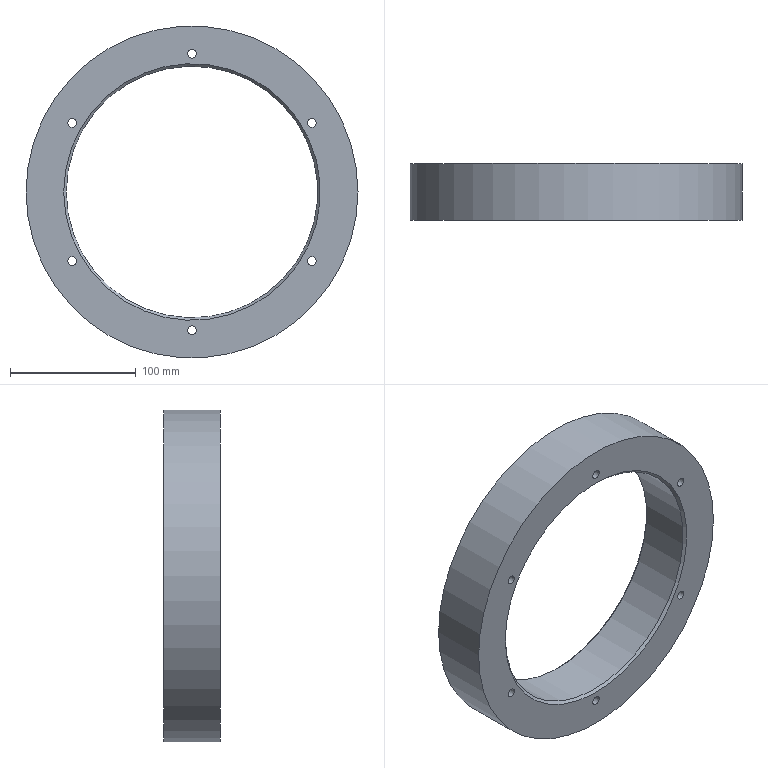Component | NX | INTERMEDIATE_CONNECTOR | 1 solid | 12 faces | box 264 x 45 x 264 mm | volume 1036622 mm3 | cylinder 8 | plane 2 | cone 2 | commonest cylinder face diameters 7 x6 264 x1 200 x1
STEP:
#1=CARTESIAN_POINT('',(0.,0.,0.));
#2=DIRECTION('',(0.,0.,1.));
#3=DIRECTION('',(1.,0.,0.));
#4=AXIS2_PLACEMENT_3D('',#1,#2,#3);
#5=CARTESIAN_POINT('',(132.,30.,-0.));
#6=VERTEX_POINT('',#5);
#7=CARTESIAN_POINT('',(-0.,30.,-0.));
#8=DIRECTION('',(0.,1.,0.));
#9=DIRECTION('',(1.,0.,0.));
#10=AXIS2_PLACEMENT_3D('',#7,#8,#9);
#11=CIRCLE('',#10,132.);
#12=CARTESIAN_POINT('',(-0.,30.,-0.));
#13=DIRECTION('',(0.,1.,0.));
#14=DIRECTION('',(-1.,0.,0.));
#15=AXIS2_PLACEMENT_3D('',#12,#13,#14);
#16=CYLINDRICAL_SURFACE('',#15,132.);
#17=CARTESIAN_POINT('',(3.142,0.));
#18=DIRECTION('',(1.,0.));
#19=VECTOR('',#18,1.);
#20=LINE('',#17,#19);
#21=(GEOMETRIC_REPRESENTATION_CONTEXT(2)PARAMETRIC_REPRESENTATION_CONTEXT()REPRESENTATION_CONTEXT('',''));
#22=DEFINITIONAL_REPRESENTATION('',(#20),#21);
#23=PCURVE('',#16,#22);
#24=CARTESIAN_POINT('',(-0.,30.,-0.));
#25=DIRECTION('',(0.,1.,0.));
#26=DIRECTION('',(-1.,0.,0.));
#27=AXIS2_PLACEMENT_3D('',#24,#25,#26);
#28=PLANE('',#27);
#29=CARTESIAN_POINT('',(0.,0.));
#30=DIRECTION('',(-1.,0.));
#31=AXIS2_PLACEMENT_2D('',#29,#30);
#32=CIRCLE('',#31,132.);
#33=(GEOMETRIC_REPRESENTATION_CONTEXT(2)PARAMETRIC_REPRESENTATION_CONTEXT()REPRESENTATION_CONTEXT('',''));
#34=DEFINITIONAL_REPRESENTATION('',(#32),#33);
#35=PCURVE('',#28,#34);
#36=SURFACE_CURVE('',#11,(#23,#35),.PCURVE_S1.);
#37=EDGE_CURVE('',#6,#6,#36,.T.);
#38=ORIENTED_EDGE('',*,*,#37,.T.);
#39=CARTESIAN_POINT('',(132.,75.,-0.));
#40=VERTEX_POINT('',#39);
#41=CARTESIAN_POINT('',(132.,30.,-0.));
#42=CARTESIAN_POINT('',(132.,75.,-0.));
#43=B_SPLINE_CURVE_WITH_KNOTS('',1,(#41,#42),.UNSPECIFIED.,.F.,.F.,(2,2),(0.,45.),.PIECEWISE_BEZIER_KNOTS.);
#44=CARTESIAN_POINT('',(9.425,0.));
#45=DIRECTION('',(0.,1.));
#46=VECTOR('',#45,1.);
#47=LINE('',#44,#46);
#48=(GEOMETRIC_REPRESENTATION_CONTEXT(2)PARAMETRIC_REPRESENTATION_CONTEXT()REPRESENTATION_CONTEXT('',''));
#49=DEFINITIONAL_REPRESENTATION('',(#47),#48);
#50=PCURVE('',#16,#49);
#51=CARTESIAN_POINT('',(3.142,0.));
#52=DIRECTION('',(0.,1.));
#53=VECTOR('',#52,1.);
#54=LINE('',#51,#53);
#55=(GEOMETRIC_REPRESENTATION_CONTEXT(2)PARAMETRIC_REPRESENTATION_CONTEXT()REPRESENTATION_CONTEXT('',''));
#56=DEFINITIONAL_REPRESENTATION('',(#54),#55);
#57=PCURVE('',#16,#56);
#58=SEAM_CURVE('',#43,(#50,#57),.PCURVE_S1.);
#59=EDGE_CURVE('',#6,#40,#58,.T.);
#60=ORIENTED_EDGE('',*,*,#59,.T.);
#61=CARTESIAN_POINT('',(-0.,75.,-0.));
#62=DIRECTION('',(0.,1.,0.));
#63=DIRECTION('',(1.,0.,0.));
#64=AXIS2_PLACEMENT_3D('',#61,#62,#63);
#65=CIRCLE('',#64,132.);
#66=CARTESIAN_POINT('',(3.142,45.));
#67=DIRECTION('',(1.,0.));
#68=VECTOR('',#67,1.);
#69=LINE('',#66,#68);
#70=(GEOMETRIC_REPRESENTATION_CONTEXT(2)PARAMETRIC_REPRESENTATION_CONTEXT()REPRESENTATION_CONTEXT('',''));
#71=DEFINITIONAL_REPRESENTATION('',(#69),#70);
#72=PCURVE('',#16,#71);
#73=CARTESIAN_POINT('',(-0.,75.,-0.));
#74=DIRECTION('',(0.,1.,0.));
#75=DIRECTION('',(-1.,0.,0.));
#76=AXIS2_PLACEMENT_3D('',#73,#74,#75);
#77=PLANE('',#76);
#78=CARTESIAN_POINT('',(0.,0.));
#79=DIRECTION('',(-1.,0.));
#80=AXIS2_PLACEMENT_2D('',#78,#79);
#81=CIRCLE('',#80,132.);
#82=(GEOMETRIC_REPRESENTATION_CONTEXT(2)PARAMETRIC_REPRESENTATION_CONTEXT()REPRESENTATION_CONTEXT('',''));
#83=DEFINITIONAL_REPRESENTATION('',(#81),#82);
#84=PCURVE('',#77,#83);
#85=SURFACE_CURVE('',#65,(#72,#84),.PCURVE_S1.);
#86=EDGE_CURVE('',#40,#40,#85,.T.);
#87=ORIENTED_EDGE('',*,*,#86,.F.);
#88=ORIENTED_EDGE('',*,*,#59,.F.);
#89=EDGE_LOOP('',(#38,#60,#87,#88));
#90=FACE_BOUND('',#89,.T.);
#91=ADVANCED_FACE('',(#90),#16,.T.);
#92=CARTESIAN_POINT('',(-100.,73.,-0.));
#93=VERTEX_POINT('',#92);
#94=CARTESIAN_POINT('',(-0.,73.,-0.));
#95=DIRECTION('',(0.,1.,0.));
#96=DIRECTION('',(-1.,0.,0.));
#97=AXIS2_PLACEMENT_3D('',#94,#95,#96);
#98=CIRCLE('',#97,100.);
#99=CARTESIAN_POINT('',(-0.,30.,-0.));
#100=DIRECTION('',(0.,1.,0.));
#101=DIRECTION('',(-1.,0.,0.));
#102=AXIS2_PLACEMENT_3D('',#99,#100,#101);
#103=CYLINDRICAL_SURFACE('',#102,100.);
#104=CARTESIAN_POINT('',(0.,43.));
#105=DIRECTION('',(1.,0.));
#106=VECTOR('',#105,1.);
#107=LINE('',#104,#106);
#108=(GEOMETRIC_REPRESENTATION_CONTEXT(2)PARAMETRIC_REPRESENTATION_CONTEXT()REPRESENTATION_CONTEXT('',''));
#109=DEFINITIONAL_REPRESENTATION('',(#107),#108);
#110=PCURVE('',#103,#109);
#111=CARTESIAN_POINT('',(-0.,73.,-0.));
#112=DIRECTION('',(0.,1.,0.));
#113=DIRECTION('',(-1.,0.,0.));
#114=AXIS2_PLACEMENT_3D('',#111,#112,#113);
#115=CONICAL_SURFACE('',#114,100.,0.7854);
#116=CARTESIAN_POINT('',(0.,0.));
#117=DIRECTION('',(1.,0.));
#118=VECTOR('',#117,1.);
#119=LINE('',#116,#118);
#120=(GEOMETRIC_REPRESENTATION_CONTEXT(2)PARAMETRIC_REPRESENTATION_CONTEXT()REPRESENTATION_CONTEXT('',''));
#121=DEFINITIONAL_REPRESENTATION('',(#119),#120);
#122=PCURVE('',#115,#121);
#123=SURFACE_CURVE('',#98,(#110,#122),.PCURVE_S1.);
#124=EDGE_CURVE('',#93,#93,#123,.T.);
#125=ORIENTED_EDGE('',*,*,#124,.F.);
#126=CARTESIAN_POINT('',(-100.,32.,-0.));
#127=VERTEX_POINT('',#126);
#128=CARTESIAN_POINT('',(-100.,32.,-0.));
#129=CARTESIAN_POINT('',(-100.,73.,-0.));
#130=B_SPLINE_CURVE_WITH_KNOTS('',1,(#128,#129),.UNSPECIFIED.,.F.,.F.,(2,2),(2.,43.),.PIECEWISE_BEZIER_KNOTS.);
#131=CARTESIAN_POINT('',(0.,0.));
#132=DIRECTION('',(0.,1.));
#133=VECTOR('',#132,1.);
#134=LINE('',#131,#133);
#135=(GEOMETRIC_REPRESENTATION_CONTEXT(2)PARAMETRIC_REPRESENTATION_CONTEXT()REPRESENTATION_CONTEXT('',''));
#136=DEFINITIONAL_REPRESENTATION('',(#134),#135);
#137=PCURVE('',#103,#136);
#138=CARTESIAN_POINT('',(6.283,0.));
#139=DIRECTION('',(0.,1.));
#140=VECTOR('',#139,1.);
#141=LINE('',#138,#140);
#142=(GEOMETRIC_REPRESENTATION_CONTEXT(2)PARAMETRIC_REPRESENTATION_CONTEXT()REPRESENTATION_CONTEXT('',''));
#143=DEFINITIONAL_REPRESENTATION('',(#141),#142);
#144=PCURVE('',#103,#143);
#145=SEAM_CURVE('',#130,(#137,#144),.PCURVE_S1.);
#146=EDGE_CURVE('',#127,#93,#145,.T.);
#147=ORIENTED_EDGE('',*,*,#146,.F.);
#148=CARTESIAN_POINT('',(-0.,32.,-0.));
#149=DIRECTION('',(0.,-1.,0.));
#150=DIRECTION('',(-1.,0.,0.));
#151=AXIS2_PLACEMENT_3D('',#148,#149,#150);
#152=CIRCLE('',#151,100.);
#153=CARTESIAN_POINT('',(6.283,2.));
#154=DIRECTION('',(-1.,0.));
#155=VECTOR('',#154,1.);
#156=LINE('',#153,#155);
#157=(GEOMETRIC_REPRESENTATION_CONTEXT(2)PARAMETRIC_REPRESENTATION_CONTEXT()REPRESENTATION_CONTEXT('',''));
#158=DEFINITIONAL_REPRESENTATION('',(#156),#157);
#159=PCURVE('',#103,#158);
#160=CARTESIAN_POINT('',(-0.,30.,-0.));
#161=DIRECTION('',(0.,-1.,0.));
#162=DIRECTION('',(1.,0.,0.));
#163=AXIS2_PLACEMENT_3D('',#160,#161,#162);
#164=CONICAL_SURFACE('',#163,102.,0.7854);
#165=CARTESIAN_POINT('',(3.142,-2.));
#166=DIRECTION('',(1.,0.));
#167=VECTOR('',#166,1.);
#168=LINE('',#165,#167);
#169=(GEOMETRIC_REPRESENTATION_CONTEXT(2)PARAMETRIC_REPRESENTATION_CONTEXT()REPRESENTATION_CONTEXT('',''));
#170=DEFINITIONAL_REPRESENTATION('',(#168),#169);
#171=PCURVE('',#164,#170);
#172=SURFACE_CURVE('',#152,(#159,#171),.PCURVE_S1.);
#173=EDGE_CURVE('',#127,#127,#172,.T.);
#174=ORIENTED_EDGE('',*,*,#173,.F.);
#175=ORIENTED_EDGE('',*,*,#146,.T.);
#176=EDGE_LOOP('',(#125,#147,#174,#175));
#177=FACE_BOUND('',#176,.F.);
#178=ADVANCED_FACE('',(#177),#103,.F.);
#179=CARTESIAN_POINT('',(-102.,30.,-0.));
#180=VERTEX_POINT('',#179);
#181=CARTESIAN_POINT('',(-0.,30.,-0.));
#182=DIRECTION('',(0.,1.,0.));
#183=DIRECTION('',(-1.,0.,0.));
#184=AXIS2_PLACEMENT_3D('',#181,#182,#183);
#185=CIRCLE('',#184,102.);
#186=CARTESIAN_POINT('',(0.,0.));
#187=DIRECTION('',(1.,0.));
#188=AXIS2_PLACEMENT_2D('',#186,#187);
#189=CIRCLE('',#188,102.);
#190=(GEOMETRIC_REPRESENTATION_CONTEXT(2)PARAMETRIC_REPRESENTATION_CONTEXT()REPRESENTATION_CONTEXT('',''));
#191=DEFINITIONAL_REPRESENTATION('',(#189),#190);
#192=PCURVE('',#28,#191);
#193=CARTESIAN_POINT('',(9.425,0.));
#194=DIRECTION('',(-1.,0.));
#195=VECTOR('',#194,1.);
#196=LINE('',#193,#195);
#197=(GEOMETRIC_REPRESENTATION_CONTEXT(2)PARAMETRIC_REPRESENTATION_CONTEXT()REPRESENTATION_CONTEXT('',''));
#198=DEFINITIONAL_REPRESENTATION('',(#196),#197);
#199=PCURVE('',#164,#198);
#200=SURFACE_CURVE('',#185,(#192,#199),.PCURVE_S1.);
#201=EDGE_CURVE('',#180,#180,#200,.T.);
#202=ORIENTED_EDGE('',*,*,#201,.T.);
#203=EDGE_LOOP('',(#202));
#204=FACE_BOUND('',#203,.T.);
#205=CARTESIAN_POINT('',(97.013,30.,51.969));
#206=VERTEX_POINT('',#205);
#207=CARTESIAN_POINT('',(95.263,30.,55.));
#208=DIRECTION('',(0.,1.,0.));
#209=DIRECTION('',(0.5,0.,-0.866));
#210=AXIS2_PLACEMENT_3D('',#207,#208,#209);
#211=CIRCLE('',#210,3.5);
#212=CARTESIAN_POINT('',(-95.263,55.));
#213=DIRECTION('',(-0.5,-0.866));
#214=AXIS2_PLACEMENT_2D('',#212,#213);
#215=CIRCLE('',#214,3.5);
#216=(GEOMETRIC_REPRESENTATION_CONTEXT(2)PARAMETRIC_REPRESENTATION_CONTEXT()REPRESENTATION_CONTEXT('',''));
#217=DEFINITIONAL_REPRESENTATION('',(#215),#216);
#218=PCURVE('',#28,#217);
#219=CARTESIAN_POINT('',(95.263,75.,55.));
#220=DIRECTION('',(0.,-1.,0.));
#221=DIRECTION('',(1.,0.,0.));
#222=AXIS2_PLACEMENT_3D('',#219,#220,#221);
#223=CYLINDRICAL_SURFACE('',#222,3.5);
#224=CARTESIAN_POINT('',(11.519,45.));
#225=DIRECTION('',(-1.,0.));
#226=VECTOR('',#225,1.);
#227=LINE('',#224,#226);
#228=(GEOMETRIC_REPRESENTATION_CONTEXT(2)PARAMETRIC_REPRESENTATION_CONTEXT()REPRESENTATION_CONTEXT('',''));
#229=DEFINITIONAL_REPRESENTATION('',(#227),#228);
#230=PCURVE('',#223,#229);
#231=SURFACE_CURVE('',#211,(#218,#230),.PCURVE_S1.);
#232=EDGE_CURVE('',#206,#206,#231,.T.);
#233=ORIENTED_EDGE('',*,*,#232,.T.);
#234=EDGE_LOOP('',(#233));
#235=FACE_BOUND('',#234,.T.);
#236=CARTESIAN_POINT('',(3.5,30.,110.));
#237=VERTEX_POINT('',#236);
#238=CARTESIAN_POINT('',(-0.,30.,110.));
#239=DIRECTION('',(0.,1.,0.));
#240=DIRECTION('',(1.,0.,0.));
#241=AXIS2_PLACEMENT_3D('',#238,#239,#240);
#242=CIRCLE('',#241,3.5);
#243=CARTESIAN_POINT('',(0.,110.));
#244=DIRECTION('',(-1.,0.));
#245=AXIS2_PLACEMENT_2D('',#243,#244);
#246=CIRCLE('',#245,3.5);
#247=(GEOMETRIC_REPRESENTATION_CONTEXT(2)PARAMETRIC_REPRESENTATION_CONTEXT()REPRESENTATION_CONTEXT('',''));
#248=DEFINITIONAL_REPRESENTATION('',(#246),#247);
#249=PCURVE('',#28,#248);
#250=CARTESIAN_POINT('',(-0.,75.,110.));
#251=DIRECTION('',(0.,-1.,0.));
#252=DIRECTION('',(1.,0.,0.));
#253=AXIS2_PLACEMENT_3D('',#250,#251,#252);
#254=CYLINDRICAL_SURFACE('',#253,3.5);
#255=CARTESIAN_POINT('',(6.283,45.));
#256=DIRECTION('',(-1.,0.));
#257=VECTOR('',#256,1.);
#258=LINE('',#255,#257);
#259=(GEOMETRIC_REPRESENTATION_CONTEXT(2)PARAMETRIC_REPRESENTATION_CONTEXT()REPRESENTATION_CONTEXT('',''));
#260=DEFINITIONAL_REPRESENTATION('',(#258),#259);
#261=PCURVE('',#254,#260);
#262=SURFACE_CURVE('',#242,(#249,#261),.PCURVE_S1.);
#263=EDGE_CURVE('',#237,#237,#262,.T.);
#264=ORIENTED_EDGE('',*,*,#263,.T.);
#265=EDGE_LOOP('',(#264));
#266=FACE_BOUND('',#265,.T.);
#267=CARTESIAN_POINT('',(-93.513,30.,58.031));
#268=VERTEX_POINT('',#267);
#269=CARTESIAN_POINT('',(-95.263,30.,55.));
#270=DIRECTION('',(0.,1.,0.));
#271=DIRECTION('',(0.5,0.,0.866));
#272=AXIS2_PLACEMENT_3D('',#269,#270,#271);
#273=CIRCLE('',#272,3.5);
#274=CARTESIAN_POINT('',(95.263,55.));
#275=DIRECTION('',(-0.5,0.866));
#276=AXIS2_PLACEMENT_2D('',#274,#275);
#277=CIRCLE('',#276,3.5);
#278=(GEOMETRIC_REPRESENTATION_CONTEXT(2)PARAMETRIC_REPRESENTATION_CONTEXT()REPRESENTATION_CONTEXT('',''));
#279=DEFINITIONAL_REPRESENTATION('',(#277),#278);
#280=PCURVE('',#28,#279);
#281=CARTESIAN_POINT('',(-95.263,75.,55.));
#282=DIRECTION('',(0.,-1.,0.));
#283=DIRECTION('',(1.,0.,0.));
#284=AXIS2_PLACEMENT_3D('',#281,#282,#283);
#285=CYLINDRICAL_SURFACE('',#284,3.5);
#286=CARTESIAN_POINT('',(7.33,45.));
#287=DIRECTION('',(-1.,0.));
#288=VECTOR('',#287,1.);
#289=LINE('',#286,#288);
#290=(GEOMETRIC_REPRESENTATION_CONTEXT(2)PARAMETRIC_REPRESENTATION_CONTEXT()REPRESENTATION_CONTEXT('',''));
#291=DEFINITIONAL_REPRESENTATION('',(#289),#290);
#292=PCURVE('',#285,#291);
#293=SURFACE_CURVE('',#273,(#280,#292),.PCURVE_S1.);
#294=EDGE_CURVE('',#268,#268,#293,.T.);
#295=ORIENTED_EDGE('',*,*,#294,.T.);
#296=EDGE_LOOP('',(#295));
#297=FACE_BOUND('',#296,.T.);
#298=CARTESIAN_POINT('',(-97.013,30.,-51.969));
#299=VERTEX_POINT('',#298);
#300=CARTESIAN_POINT('',(-95.263,30.,-55.));
#301=DIRECTION('',(0.,1.,0.));
#302=DIRECTION('',(-0.5,0.,0.866));
#303=AXIS2_PLACEMENT_3D('',#300,#301,#302);
#304=CIRCLE('',#303,3.5);
#305=CARTESIAN_POINT('',(95.263,-55.));
#306=DIRECTION('',(0.5,0.866));
#307=AXIS2_PLACEMENT_2D('',#305,#306);
#308=CIRCLE('',#307,3.5);
#309=(GEOMETRIC_REPRESENTATION_CONTEXT(2)PARAMETRIC_REPRESENTATION_CONTEXT()REPRESENTATION_CONTEXT('',''));
#310=DEFINITIONAL_REPRESENTATION('',(#308),#309);
#311=PCURVE('',#28,#310);
#312=CARTESIAN_POINT('',(-95.263,75.,-55.));
#313=DIRECTION('',(0.,-1.,0.));
#314=DIRECTION('',(1.,0.,0.));
#315=AXIS2_PLACEMENT_3D('',#312,#313,#314);
#316=CYLINDRICAL_SURFACE('',#315,3.5);
#317=CARTESIAN_POINT('',(8.378,45.));
#318=DIRECTION('',(-1.,0.));
#319=VECTOR('',#318,1.);
#320=LINE('',#317,#319);
#321=(GEOMETRIC_REPRESENTATION_CONTEXT(2)PARAMETRIC_REPRESENTATION_CONTEXT()REPRESENTATION_CONTEXT('',''));
#322=DEFINITIONAL_REPRESENTATION('',(#320),#321);
#323=PCURVE('',#316,#322);
#324=SURFACE_CURVE('',#304,(#311,#323),.PCURVE_S1.);
#325=EDGE_CURVE('',#299,#299,#324,.T.);
#326=ORIENTED_EDGE('',*,*,#325,.T.);
#327=EDGE_LOOP('',(#326));
#328=FACE_BOUND('',#327,.T.);
#329=CARTESIAN_POINT('',(-3.5,30.,-110.));
#330=VERTEX_POINT('',#329);
#331=CARTESIAN_POINT('',(-0.,30.,-110.));
#332=DIRECTION('',(0.,1.,0.));
#333=DIRECTION('',(-1.,0.,0.));
#334=AXIS2_PLACEMENT_3D('',#331,#332,#333);
#335=CIRCLE('',#334,3.5);
#336=CARTESIAN_POINT('',(0.,-110.));
#337=DIRECTION('',(1.,0.));
#338=AXIS2_PLACEMENT_2D('',#336,#337);
#339=CIRCLE('',#338,3.5);
#340=(GEOMETRIC_REPRESENTATION_CONTEXT(2)PARAMETRIC_REPRESENTATION_CONTEXT()REPRESENTATION_CONTEXT('',''));
#341=DEFINITIONAL_REPRESENTATION('',(#339),#340);
#342=PCURVE('',#28,#341);
#343=CARTESIAN_POINT('',(-0.,75.,-110.));
#344=DIRECTION('',(0.,-1.,0.));
#345=DIRECTION('',(1.,0.,0.));
#346=AXIS2_PLACEMENT_3D('',#343,#344,#345);
#347=CYLINDRICAL_SURFACE('',#346,3.5);
#348=CARTESIAN_POINT('',(9.425,45.));
#349=DIRECTION('',(-1.,0.));
#350=VECTOR('',#349,1.);
#351=LINE('',#348,#350);
#352=(GEOMETRIC_REPRESENTATION_CONTEXT(2)PARAMETRIC_REPRESENTATION_CONTEXT()REPRESENTATION_CONTEXT('',''));
#353=DEFINITIONAL_REPRESENTATION('',(#351),#352);
#354=PCURVE('',#347,#353);
#355=SURFACE_CURVE('',#335,(#342,#354),.PCURVE_S1.);
#356=EDGE_CURVE('',#330,#330,#355,.T.);
#357=ORIENTED_EDGE('',*,*,#356,.T.);
#358=EDGE_LOOP('',(#357));
#359=FACE_BOUND('',#358,.T.);
#360=CARTESIAN_POINT('',(93.513,30.,-58.031));
#361=VERTEX_POINT('',#360);
#362=CARTESIAN_POINT('',(95.263,30.,-55.));
#363=DIRECTION('',(0.,1.,0.));
#364=DIRECTION('',(-0.5,0.,-0.866));
#365=AXIS2_PLACEMENT_3D('',#362,#363,#364);
#366=CIRCLE('',#365,3.5);
#367=CARTESIAN_POINT('',(-95.263,-55.));
#368=DIRECTION('',(0.5,-0.866));
#369=AXIS2_PLACEMENT_2D('',#367,#368);
#370=CIRCLE('',#369,3.5);
#371=(GEOMETRIC_REPRESENTATION_CONTEXT(2)PARAMETRIC_REPRESENTATION_CONTEXT()REPRESENTATION_CONTEXT('',''));
#372=DEFINITIONAL_REPRESENTATION('',(#370),#371);
#373=PCURVE('',#28,#372);
#374=CARTESIAN_POINT('',(95.263,75.,-55.));
#375=DIRECTION('',(0.,-1.,0.));
#376=DIRECTION('',(1.,0.,0.));
#377=AXIS2_PLACEMENT_3D('',#374,#375,#376);
#378=CYLINDRICAL_SURFACE('',#377,3.5);
#379=CARTESIAN_POINT('',(10.472,45.));
#380=DIRECTION('',(-1.,0.));
#381=VECTOR('',#380,1.);
#382=LINE('',#379,#381);
#383=(GEOMETRIC_REPRESENTATION_CONTEXT(2)PARAMETRIC_REPRESENTATION_CONTEXT()REPRESENTATION_CONTEXT('',''));
#384=DEFINITIONAL_REPRESENTATION('',(#382),#383);
#385=PCURVE('',#378,#384);
#386=SURFACE_CURVE('',#366,(#373,#385),.PCURVE_S1.);
#387=EDGE_CURVE('',#361,#361,#386,.T.);
#388=ORIENTED_EDGE('',*,*,#387,.T.);
#389=EDGE_LOOP('',(#388));
#390=FACE_BOUND('',#389,.T.);
#391=ORIENTED_EDGE('',*,*,#37,.F.);
#392=EDGE_LOOP('',(#391));
#393=FACE_BOUND('',#392,.T.);
#394=ADVANCED_FACE('',(#204,#235,#266,#297,#328,#359,#390,#393),#28,.F.);
#395=CARTESIAN_POINT('',(-102.,75.,-0.));
#396=VERTEX_POINT('',#395);
#397=CARTESIAN_POINT('',(-0.,75.,-0.));
#398=DIRECTION('',(0.,-1.,0.));
#399=DIRECTION('',(-1.,0.,0.));
#400=AXIS2_PLACEMENT_3D('',#397,#398,#399);
#401=CIRCLE('',#400,102.);
#402=CARTESIAN_POINT('',(102.,0.));
#403=CARTESIAN_POINT('',(102.,-176.669));
#404=CARTESIAN_POINT('',(-51.,-88.335));
#405=CARTESIAN_POINT('',(-204.,-0.));
#406=CARTESIAN_POINT('',(-51.,88.335));
#407=CARTESIAN_POINT('',(102.,176.669));
#408=CARTESIAN_POINT('',(102.,0.));
#409=(BOUNDED_CURVE()B_SPLINE_CURVE(2,(#402,#403,#404,#405,#406,#407,#408),.UNSPECIFIED.,.T.,.F.)B_SPLINE_CURVE_WITH_KNOTS((1,2,2,2,2,1),(-2.094,0.,2.094,4.189,6.283,8.378),.UNSPECIFIED.)CURVE()GEOMETRIC_REPRESENTATION_ITEM()RATIONAL_B_SPLINE_CURVE((1.,0.5,1.,0.5,1.,0.5,1.))REPRESENTATION_ITEM(''));
#410=(GEOMETRIC_REPRESENTATION_CONTEXT(2)PARAMETRIC_REPRESENTATION_CONTEXT()REPRESENTATION_CONTEXT('',''));
#411=DEFINITIONAL_REPRESENTATION('',(#409),#410);
#412=PCURVE('',#77,#411);
#413=CARTESIAN_POINT('',(6.283,2.));
#414=DIRECTION('',(-1.,0.));
#415=VECTOR('',#414,1.);
#416=LINE('',#413,#415);
#417=(GEOMETRIC_REPRESENTATION_CONTEXT(2)PARAMETRIC_REPRESENTATION_CONTEXT()REPRESENTATION_CONTEXT('',''));
#418=DEFINITIONAL_REPRESENTATION('',(#416),#417);
#419=PCURVE('',#115,#418);
#420=SURFACE_CURVE('',#401,(#412,#419),.PCURVE_S1.);
#421=EDGE_CURVE('',#396,#396,#420,.T.);
#422=ORIENTED_EDGE('',*,*,#421,.T.);
#423=EDGE_LOOP('',(#422));
#424=FACE_BOUND('',#423,.T.);
#425=CARTESIAN_POINT('',(97.013,75.,51.969));
#426=VERTEX_POINT('',#425);
#427=CARTESIAN_POINT('',(95.263,75.,55.));
#428=DIRECTION('',(0.,1.,0.));
#429=DIRECTION('',(0.5,0.,-0.866));
#430=AXIS2_PLACEMENT_3D('',#427,#428,#429);
#431=CIRCLE('',#430,3.5);
#432=CARTESIAN_POINT('',(-95.263,55.));
#433=DIRECTION('',(-0.5,-0.866));
#434=AXIS2_PLACEMENT_2D('',#432,#433);
#435=CIRCLE('',#434,3.5);
#436=(GEOMETRIC_REPRESENTATION_CONTEXT(2)PARAMETRIC_REPRESENTATION_CONTEXT()REPRESENTATION_CONTEXT('',''));
#437=DEFINITIONAL_REPRESENTATION('',(#435),#436);
#438=PCURVE('',#77,#437);
#439=CARTESIAN_POINT('',(11.519,0.));
#440=DIRECTION('',(-1.,0.));
#441=VECTOR('',#440,1.);
#442=LINE('',#439,#441);
#443=(GEOMETRIC_REPRESENTATION_CONTEXT(2)PARAMETRIC_REPRESENTATION_CONTEXT()REPRESENTATION_CONTEXT('',''));
#444=DEFINITIONAL_REPRESENTATION('',(#442),#443);
#445=PCURVE('',#223,#444);
#446=SURFACE_CURVE('',#431,(#438,#445),.PCURVE_S1.);
#447=EDGE_CURVE('',#426,#426,#446,.T.);
#448=ORIENTED_EDGE('',*,*,#447,.F.);
#449=EDGE_LOOP('',(#448));
#450=FACE_BOUND('',#449,.T.);
#451=CARTESIAN_POINT('',(3.5,75.,110.));
#452=VERTEX_POINT('',#451);
#453=CARTESIAN_POINT('',(-0.,75.,110.));
#454=DIRECTION('',(0.,1.,0.));
#455=DIRECTION('',(1.,0.,0.));
#456=AXIS2_PLACEMENT_3D('',#453,#454,#455);
#457=CIRCLE('',#456,3.5);
#458=CARTESIAN_POINT('',(0.,110.));
#459=DIRECTION('',(-1.,0.));
#460=AXIS2_PLACEMENT_2D('',#458,#459);
#461=CIRCLE('',#460,3.5);
#462=(GEOMETRIC_REPRESENTATION_CONTEXT(2)PARAMETRIC_REPRESENTATION_CONTEXT()REPRESENTATION_CONTEXT('',''));
#463=DEFINITIONAL_REPRESENTATION('',(#461),#462);
#464=PCURVE('',#77,#463);
#465=CARTESIAN_POINT('',(6.283,0.));
#466=DIRECTION('',(-1.,0.));
#467=VECTOR('',#466,1.);
#468=LINE('',#465,#467);
#469=(GEOMETRIC_REPRESENTATION_CONTEXT(2)PARAMETRIC_REPRESENTATION_CONTEXT()REPRESENTATION_CONTEXT('',''));
#470=DEFINITIONAL_REPRESENTATION('',(#468),#469);
#471=PCURVE('',#254,#470);
#472=SURFACE_CURVE('',#457,(#464,#471),.PCURVE_S1.);
#473=EDGE_CURVE('',#452,#452,#472,.T.);
#474=ORIENTED_EDGE('',*,*,#473,.F.);
#475=EDGE_LOOP('',(#474));
#476=FACE_BOUND('',#475,.T.);
#477=CARTESIAN_POINT('',(-93.513,75.,58.031));
#478=VERTEX_POINT('',#477);
#479=CARTESIAN_POINT('',(-95.263,75.,55.));
#480=DIRECTION('',(0.,1.,0.));
#481=DIRECTION('',(0.5,0.,0.866));
#482=AXIS2_PLACEMENT_3D('',#479,#480,#481);
#483=CIRCLE('',#482,3.5);
#484=CARTESIAN_POINT('',(95.263,55.));
#485=DIRECTION('',(-0.5,0.866));
#486=AXIS2_PLACEMENT_2D('',#484,#485);
#487=CIRCLE('',#486,3.5);
#488=(GEOMETRIC_REPRESENTATION_CONTEXT(2)PARAMETRIC_REPRESENTATION_CONTEXT()REPRESENTATION_CONTEXT('',''));
#489=DEFINITIONAL_REPRESENTATION('',(#487),#488);
#490=PCURVE('',#77,#489);
#491=CARTESIAN_POINT('',(7.33,0.));
#492=DIRECTION('',(-1.,0.));
#493=VECTOR('',#492,1.);
#494=LINE('',#491,#493);
#495=(GEOMETRIC_REPRESENTATION_CONTEXT(2)PARAMETRIC_REPRESENTATION_CONTEXT()REPRESENTATION_CONTEXT('',''));
#496=DEFINITIONAL_REPRESENTATION('',(#494),#495);
#497=PCURVE('',#285,#496);
#498=SURFACE_CURVE('',#483,(#490,#497),.PCURVE_S1.);
#499=EDGE_CURVE('',#478,#478,#498,.T.);
#500=ORIENTED_EDGE('',*,*,#499,.F.);
#501=EDGE_LOOP('',(#500));
#502=FACE_BOUND('',#501,.T.);
#503=CARTESIAN_POINT('',(-97.013,75.,-51.969));
#504=VERTEX_POINT('',#503);
#505=CARTESIAN_POINT('',(-95.263,75.,-55.));
#506=DIRECTION('',(0.,1.,0.));
#507=DIRECTION('',(-0.5,0.,0.866));
#508=AXIS2_PLACEMENT_3D('',#505,#506,#507);
#509=CIRCLE('',#508,3.5);
#510=CARTESIAN_POINT('',(95.263,-55.));
#511=DIRECTION('',(0.5,0.866));
#512=AXIS2_PLACEMENT_2D('',#510,#511);
#513=CIRCLE('',#512,3.5);
#514=(GEOMETRIC_REPRESENTATION_CONTEXT(2)PARAMETRIC_REPRESENTATION_CONTEXT()REPRESENTATION_CONTEXT('',''));
#515=DEFINITIONAL_REPRESENTATION('',(#513),#514);
#516=PCURVE('',#77,#515);
#517=CARTESIAN_POINT('',(8.378,0.));
#518=DIRECTION('',(-1.,0.));
#519=VECTOR('',#518,1.);
#520=LINE('',#517,#519);
#521=(GEOMETRIC_REPRESENTATION_CONTEXT(2)PARAMETRIC_REPRESENTATION_CONTEXT()REPRESENTATION_CONTEXT('',''));
#522=DEFINITIONAL_REPRESENTATION('',(#520),#521);
#523=PCURVE('',#316,#522);
#524=SURFACE_CURVE('',#509,(#516,#523),.PCURVE_S1.);
#525=EDGE_CURVE('',#504,#504,#524,.T.);
#526=ORIENTED_EDGE('',*,*,#525,.F.);
#527=EDGE_LOOP('',(#526));
#528=FACE_BOUND('',#527,.T.);
#529=CARTESIAN_POINT('',(-3.5,75.,-110.));
#530=VERTEX_POINT('',#529);
#531=CARTESIAN_POINT('',(-0.,75.,-110.));
#532=DIRECTION('',(0.,1.,0.));
#533=DIRECTION('',(-1.,0.,0.));
#534=AXIS2_PLACEMENT_3D('',#531,#532,#533);
#535=CIRCLE('',#534,3.5);
#536=CARTESIAN_POINT('',(0.,-110.));
#537=DIRECTION('',(1.,0.));
#538=AXIS2_PLACEMENT_2D('',#536,#537);
#539=CIRCLE('',#538,3.5);
#540=(GEOMETRIC_REPRESENTATION_CONTEXT(2)PARAMETRIC_REPRESENTATION_CONTEXT()REPRESENTATION_CONTEXT('',''));
#541=DEFINITIONAL_REPRESENTATION('',(#539),#540);
#542=PCURVE('',#77,#541);
#543=CARTESIAN_POINT('',(9.425,0.));
#544=DIRECTION('',(-1.,0.));
#545=VECTOR('',#544,1.);
#546=LINE('',#543,#545);
#547=(GEOMETRIC_REPRESENTATION_CONTEXT(2)PARAMETRIC_REPRESENTATION_CONTEXT()REPRESENTATION_CONTEXT('',''));
#548=DEFINITIONAL_REPRESENTATION('',(#546),#547);
#549=PCURVE('',#347,#548);
#550=SURFACE_CURVE('',#535,(#542,#549),.PCURVE_S1.);
#551=EDGE_CURVE('',#530,#530,#550,.T.);
#552=ORIENTED_EDGE('',*,*,#551,.F.);
#553=EDGE_LOOP('',(#552));
#554=FACE_BOUND('',#553,.T.);
#555=CARTESIAN_POINT('',(93.513,75.,-58.031));
#556=VERTEX_POINT('',#555);
#557=CARTESIAN_POINT('',(95.263,75.,-55.));
#558=DIRECTION('',(0.,1.,0.));
#559=DIRECTION('',(-0.5,0.,-0.866));
#560=AXIS2_PLACEMENT_3D('',#557,#558,#559);
#561=CIRCLE('',#560,3.5);
#562=CARTESIAN_POINT('',(-95.263,-55.));
#563=DIRECTION('',(0.5,-0.866));
#564=AXIS2_PLACEMENT_2D('',#562,#563);
#565=CIRCLE('',#564,3.5);
#566=(GEOMETRIC_REPRESENTATION_CONTEXT(2)PARAMETRIC_REPRESENTATION_CONTEXT()REPRESENTATION_CONTEXT('',''));
#567=DEFINITIONAL_REPRESENTATION('',(#565),#566);
#568=PCURVE('',#77,#567);
#569=CARTESIAN_POINT('',(10.472,0.));
#570=DIRECTION('',(-1.,0.));
#571=VECTOR('',#570,1.);
#572=LINE('',#569,#571);
#573=(GEOMETRIC_REPRESENTATION_CONTEXT(2)PARAMETRIC_REPRESENTATION_CONTEXT()REPRESENTATION_CONTEXT('',''));
#574=DEFINITIONAL_REPRESENTATION('',(#572),#573);
#575=PCURVE('',#378,#574);
#576=SURFACE_CURVE('',#561,(#568,#575),.PCURVE_S1.);
#577=EDGE_CURVE('',#556,#556,#576,.T.);
#578=ORIENTED_EDGE('',*,*,#577,.F.);
#579=EDGE_LOOP('',(#578));
#580=FACE_BOUND('',#579,.T.);
#581=ORIENTED_EDGE('',*,*,#86,.T.);
#582=EDGE_LOOP('',(#581));
#583=FACE_BOUND('',#582,.T.);
#584=ADVANCED_FACE('',(#424,#450,#476,#502,#528,#554,#580,#583),#77,.T.);
#585=ORIENTED_EDGE('',*,*,#577,.F.);
#586=CARTESIAN_POINT('',(93.513,75.,-58.031));
#587=CARTESIAN_POINT('',(93.513,30.,-58.031));
#588=B_SPLINE_CURVE_WITH_KNOTS('',1,(#586,#587),.UNSPECIFIED.,.F.,.F.,(2,2),(0.,45.),.PIECEWISE_BEZIER_KNOTS.);
#589=CARTESIAN_POINT('',(10.472,0.));
#590=DIRECTION('',(0.,1.));
#591=VECTOR('',#590,1.);
#592=LINE('',#589,#591);
#593=(GEOMETRIC_REPRESENTATION_CONTEXT(2)PARAMETRIC_REPRESENTATION_CONTEXT()REPRESENTATION_CONTEXT('',''));
#594=DEFINITIONAL_REPRESENTATION('',(#592),#593);
#595=PCURVE('',#378,#594);
#596=CARTESIAN_POINT('',(4.189,0.));
#597=DIRECTION('',(0.,1.));
#598=VECTOR('',#597,1.);
#599=LINE('',#596,#598);
#600=(GEOMETRIC_REPRESENTATION_CONTEXT(2)PARAMETRIC_REPRESENTATION_CONTEXT()REPRESENTATION_CONTEXT('',''));
#601=DEFINITIONAL_REPRESENTATION('',(#599),#600);
#602=PCURVE('',#378,#601);
#603=SEAM_CURVE('',#588,(#595,#602),.PCURVE_S1.);
#604=EDGE_CURVE('',#556,#361,#603,.T.);
#605=ORIENTED_EDGE('',*,*,#604,.T.);
#606=ORIENTED_EDGE('',*,*,#387,.T.);
#607=ORIENTED_EDGE('',*,*,#604,.F.);
#608=EDGE_LOOP('',(#585,#605,#606,#607));
#609=FACE_BOUND('',#608,.F.);
#610=ADVANCED_FACE('',(#609),#378,.F.);
#611=ORIENTED_EDGE('',*,*,#551,.F.);
#612=CARTESIAN_POINT('',(-3.5,75.,-110.));
#613=CARTESIAN_POINT('',(-3.5,30.,-110.));
#614=B_SPLINE_CURVE_WITH_KNOTS('',1,(#612,#613),.UNSPECIFIED.,.F.,.F.,(2,2),(0.,45.),.PIECEWISE_BEZIER_KNOTS.);
#615=CARTESIAN_POINT('',(9.425,0.));
#616=DIRECTION('',(0.,1.));
#617=VECTOR('',#616,1.);
#618=LINE('',#615,#617);
#619=(GEOMETRIC_REPRESENTATION_CONTEXT(2)PARAMETRIC_REPRESENTATION_CONTEXT()REPRESENTATION_CONTEXT('',''));
#620=DEFINITIONAL_REPRESENTATION('',(#618),#619);
#621=PCURVE('',#347,#620);
#622=CARTESIAN_POINT('',(3.142,0.));
#623=DIRECTION('',(0.,1.));
#624=VECTOR('',#623,1.);
#625=LINE('',#622,#624);
#626=(GEOMETRIC_REPRESENTATION_CONTEXT(2)PARAMETRIC_REPRESENTATION_CONTEXT()REPRESENTATION_CONTEXT('',''));
#627=DEFINITIONAL_REPRESENTATION('',(#625),#626);
#628=PCURVE('',#347,#627);
#629=SEAM_CURVE('',#614,(#621,#628),.PCURVE_S1.);
#630=EDGE_CURVE('',#530,#330,#629,.T.);
#631=ORIENTED_EDGE('',*,*,#630,.T.);
#632=ORIENTED_EDGE('',*,*,#356,.T.);
#633=ORIENTED_EDGE('',*,*,#630,.F.);
#634=EDGE_LOOP('',(#611,#631,#632,#633));
#635=FACE_BOUND('',#634,.F.);
#636=ADVANCED_FACE('',(#635),#347,.F.);
#637=ORIENTED_EDGE('',*,*,#525,.F.);
#638=CARTESIAN_POINT('',(-97.013,75.,-51.969));
#639=CARTESIAN_POINT('',(-97.013,30.,-51.969));
#640=B_SPLINE_CURVE_WITH_KNOTS('',1,(#638,#639),.UNSPECIFIED.,.F.,.F.,(2,2),(0.,45.),.PIECEWISE_BEZIER_KNOTS.);
#641=CARTESIAN_POINT('',(8.378,0.));
#642=DIRECTION('',(0.,1.));
#643=VECTOR('',#642,1.);
#644=LINE('',#641,#643);
#645=(GEOMETRIC_REPRESENTATION_CONTEXT(2)PARAMETRIC_REPRESENTATION_CONTEXT()REPRESENTATION_CONTEXT('',''));
#646=DEFINITIONAL_REPRESENTATION('',(#644),#645);
#647=PCURVE('',#316,#646);
#648=CARTESIAN_POINT('',(2.094,0.));
#649=DIRECTION('',(0.,1.));
#650=VECTOR('',#649,1.);
#651=LINE('',#648,#650);
#652=(GEOMETRIC_REPRESENTATION_CONTEXT(2)PARAMETRIC_REPRESENTATION_CONTEXT()REPRESENTATION_CONTEXT('',''));
#653=DEFINITIONAL_REPRESENTATION('',(#651),#652);
#654=PCURVE('',#316,#653);
#655=SEAM_CURVE('',#640,(#647,#654),.PCURVE_S1.);
#656=EDGE_CURVE('',#504,#299,#655,.T.);
#657=ORIENTED_EDGE('',*,*,#656,.T.);
#658=ORIENTED_EDGE('',*,*,#325,.T.);
#659=ORIENTED_EDGE('',*,*,#656,.F.);
#660=EDGE_LOOP('',(#637,#657,#658,#659));
#661=FACE_BOUND('',#660,.F.);
#662=ADVANCED_FACE('',(#661),#316,.F.);
#663=ORIENTED_EDGE('',*,*,#499,.F.);
#664=CARTESIAN_POINT('',(-93.513,75.,58.031));
#665=CARTESIAN_POINT('',(-93.513,30.,58.031));
#666=B_SPLINE_CURVE_WITH_KNOTS('',1,(#664,#665),.UNSPECIFIED.,.F.,.F.,(2,2),(0.,45.),.PIECEWISE_BEZIER_KNOTS.);
#667=CARTESIAN_POINT('',(7.33,0.));
#668=DIRECTION('',(0.,1.));
#669=VECTOR('',#668,1.);
#670=LINE('',#667,#669);
#671=(GEOMETRIC_REPRESENTATION_CONTEXT(2)PARAMETRIC_REPRESENTATION_CONTEXT()REPRESENTATION_CONTEXT('',''));
#672=DEFINITIONAL_REPRESENTATION('',(#670),#671);
#673=PCURVE('',#285,#672);
#674=CARTESIAN_POINT('',(1.047,0.));
#675=DIRECTION('',(0.,1.));
#676=VECTOR('',#675,1.);
#677=LINE('',#674,#676);
#678=(GEOMETRIC_REPRESENTATION_CONTEXT(2)PARAMETRIC_REPRESENTATION_CONTEXT()REPRESENTATION_CONTEXT('',''));
#679=DEFINITIONAL_REPRESENTATION('',(#677),#678);
#680=PCURVE('',#285,#679);
#681=SEAM_CURVE('',#666,(#673,#680),.PCURVE_S1.);
#682=EDGE_CURVE('',#478,#268,#681,.T.);
#683=ORIENTED_EDGE('',*,*,#682,.T.);
#684=ORIENTED_EDGE('',*,*,#294,.T.);
#685=ORIENTED_EDGE('',*,*,#682,.F.);
#686=EDGE_LOOP('',(#663,#683,#684,#685));
#687=FACE_BOUND('',#686,.F.);
#688=ADVANCED_FACE('',(#687),#285,.F.);
#689=ORIENTED_EDGE('',*,*,#473,.F.);
#690=CARTESIAN_POINT('',(3.5,75.,110.));
#691=CARTESIAN_POINT('',(3.5,30.,110.));
#692=B_SPLINE_CURVE_WITH_KNOTS('',1,(#690,#691),.UNSPECIFIED.,.F.,.F.,(2,2),(0.,45.),.PIECEWISE_BEZIER_KNOTS.);
#693=CARTESIAN_POINT('',(6.283,0.));
#694=DIRECTION('',(0.,1.));
#695=VECTOR('',#694,1.);
#696=LINE('',#693,#695);
#697=(GEOMETRIC_REPRESENTATION_CONTEXT(2)PARAMETRIC_REPRESENTATION_CONTEXT()REPRESENTATION_CONTEXT('',''));
#698=DEFINITIONAL_REPRESENTATION('',(#696),#697);
#699=PCURVE('',#254,#698);
#700=CARTESIAN_POINT('',(0.,0.));
#701=DIRECTION('',(0.,1.));
#702=VECTOR('',#701,1.);
#703=LINE('',#700,#702);
#704=(GEOMETRIC_REPRESENTATION_CONTEXT(2)PARAMETRIC_REPRESENTATION_CONTEXT()REPRESENTATION_CONTEXT('',''));
#705=DEFINITIONAL_REPRESENTATION('',(#703),#704);
#706=PCURVE('',#254,#705);
#707=SEAM_CURVE('',#692,(#699,#706),.PCURVE_S1.);
#708=EDGE_CURVE('',#452,#237,#707,.T.);
#709=ORIENTED_EDGE('',*,*,#708,.T.);
#710=ORIENTED_EDGE('',*,*,#263,.T.);
#711=ORIENTED_EDGE('',*,*,#708,.F.);
#712=EDGE_LOOP('',(#689,#709,#710,#711));
#713=FACE_BOUND('',#712,.F.);
#714=ADVANCED_FACE('',(#713),#254,.F.);
#715=ORIENTED_EDGE('',*,*,#447,.F.);
#716=CARTESIAN_POINT('',(97.013,75.,51.969));
#717=CARTESIAN_POINT('',(97.013,30.,51.969));
#718=B_SPLINE_CURVE_WITH_KNOTS('',1,(#716,#717),.UNSPECIFIED.,.F.,.F.,(2,2),(0.,45.),.PIECEWISE_BEZIER_KNOTS.);
#719=CARTESIAN_POINT('',(11.519,0.));
#720=DIRECTION('',(0.,1.));
#721=VECTOR('',#720,1.);
#722=LINE('',#719,#721);
#723=(GEOMETRIC_REPRESENTATION_CONTEXT(2)PARAMETRIC_REPRESENTATION_CONTEXT()REPRESENTATION_CONTEXT('',''));
#724=DEFINITIONAL_REPRESENTATION('',(#722),#723);
#725=PCURVE('',#223,#724);
#726=CARTESIAN_POINT('',(5.236,0.));
#727=DIRECTION('',(0.,1.));
#728=VECTOR('',#727,1.);
#729=LINE('',#726,#728);
#730=(GEOMETRIC_REPRESENTATION_CONTEXT(2)PARAMETRIC_REPRESENTATION_CONTEXT()REPRESENTATION_CONTEXT('',''));
#731=DEFINITIONAL_REPRESENTATION('',(#729),#730);
#732=PCURVE('',#223,#731);
#733=SEAM_CURVE('',#718,(#725,#732),.PCURVE_S1.);
#734=EDGE_CURVE('',#426,#206,#733,.T.);
#735=ORIENTED_EDGE('',*,*,#734,.T.);
#736=ORIENTED_EDGE('',*,*,#232,.T.);
#737=ORIENTED_EDGE('',*,*,#734,.F.);
#738=EDGE_LOOP('',(#715,#735,#736,#737));
#739=FACE_BOUND('',#738,.F.);
#740=ADVANCED_FACE('',(#739),#223,.F.);
#741=ORIENTED_EDGE('',*,*,#421,.T.);
#742=CARTESIAN_POINT('',(-100.,73.,-0.));
#743=CARTESIAN_POINT('',(-102.,75.,-0.));
#744=B_SPLINE_CURVE_WITH_KNOTS('',1,(#742,#743),.UNSPECIFIED.,.F.,.F.,(2,2),(0.,2.828),.PIECEWISE_BEZIER_KNOTS.);
#745=CARTESIAN_POINT('',(0.,0.));
#746=DIRECTION('',(0.,1.));
#747=VECTOR('',#746,1.);
#748=LINE('',#745,#747);
#749=(GEOMETRIC_REPRESENTATION_CONTEXT(2)PARAMETRIC_REPRESENTATION_CONTEXT()REPRESENTATION_CONTEXT('',''));
#750=DEFINITIONAL_REPRESENTATION('',(#748),#749);
#751=PCURVE('',#115,#750);
#752=CARTESIAN_POINT('',(6.283,0.));
#753=DIRECTION('',(0.,1.));
#754=VECTOR('',#753,1.);
#755=LINE('',#752,#754);
#756=(GEOMETRIC_REPRESENTATION_CONTEXT(2)PARAMETRIC_REPRESENTATION_CONTEXT()REPRESENTATION_CONTEXT('',''));
#757=DEFINITIONAL_REPRESENTATION('',(#755),#756);
#758=PCURVE('',#115,#757);
#759=SEAM_CURVE('',#744,(#751,#758),.PCURVE_S1.);
#760=EDGE_CURVE('',#93,#396,#759,.T.);
#761=ORIENTED_EDGE('',*,*,#760,.F.);
#762=ORIENTED_EDGE('',*,*,#124,.T.);
#763=ORIENTED_EDGE('',*,*,#760,.T.);
#764=EDGE_LOOP('',(#741,#761,#762,#763));
#765=FACE_BOUND('',#764,.F.);
#766=ADVANCED_FACE('',(#765),#115,.F.);
#767=ORIENTED_EDGE('',*,*,#173,.T.);
#768=CARTESIAN_POINT('',(-100.,32.,-0.));
#769=CARTESIAN_POINT('',(-102.,30.,-0.));
#770=B_SPLINE_CURVE_WITH_KNOTS('',1,(#768,#769),.UNSPECIFIED.,.F.,.F.,(2,2),(-2.828,0.),.PIECEWISE_BEZIER_KNOTS.);
#771=CARTESIAN_POINT('',(9.425,0.));
#772=DIRECTION('',(0.,1.));
#773=VECTOR('',#772,1.);
#774=LINE('',#771,#773);
#775=(GEOMETRIC_REPRESENTATION_CONTEXT(2)PARAMETRIC_REPRESENTATION_CONTEXT()REPRESENTATION_CONTEXT('',''));
#776=DEFINITIONAL_REPRESENTATION('',(#774),#775);
#777=PCURVE('',#164,#776);
#778=CARTESIAN_POINT('',(3.142,0.));
#779=DIRECTION('',(0.,1.));
#780=VECTOR('',#779,1.);
#781=LINE('',#778,#780);
#782=(GEOMETRIC_REPRESENTATION_CONTEXT(2)PARAMETRIC_REPRESENTATION_CONTEXT()REPRESENTATION_CONTEXT('',''));
#783=DEFINITIONAL_REPRESENTATION('',(#781),#782);
#784=PCURVE('',#164,#783);
#785=SEAM_CURVE('',#770,(#777,#784),.PCURVE_S1.);
#786=EDGE_CURVE('',#127,#180,#785,.T.);
#787=ORIENTED_EDGE('',*,*,#786,.T.);
#788=ORIENTED_EDGE('',*,*,#201,.T.);
#789=ORIENTED_EDGE('',*,*,#786,.F.);
#790=EDGE_LOOP('',(#767,#787,#788,#789));
#791=FACE_BOUND('',#790,.F.);
#792=ADVANCED_FACE('',(#791),#164,.F.);
#793=CLOSED_SHELL('',(#91,#178,#394,#584,#610,#636,#662,#688,#714,#740,#766,#792));
#794=MANIFOLD_SOLID_BREP('',#793);
#795=(LENGTH_UNIT()NAMED_UNIT(*)SI_UNIT(.MILLI.,.METRE.));
#796=UNCERTAINTY_MEASURE_WITH_UNIT(LENGTH_MEASURE(0.00001),#795,'','');
#797=(NAMED_UNIT(*)PLANE_ANGLE_UNIT()SI_UNIT($,.RADIAN.));
#798=(NAMED_UNIT(*)SI_UNIT($,.STERADIAN.)SOLID_ANGLE_UNIT());
#799=(GEOMETRIC_REPRESENTATION_CONTEXT(3)GLOBAL_UNCERTAINTY_ASSIGNED_CONTEXT((#796))GLOBAL_UNIT_ASSIGNED_CONTEXT((#795,#797,#798))REPRESENTATION_CONTEXT('',''));
#800=ADVANCED_BREP_SHAPE_REPRESENTATION('',(#4,#794),#799);